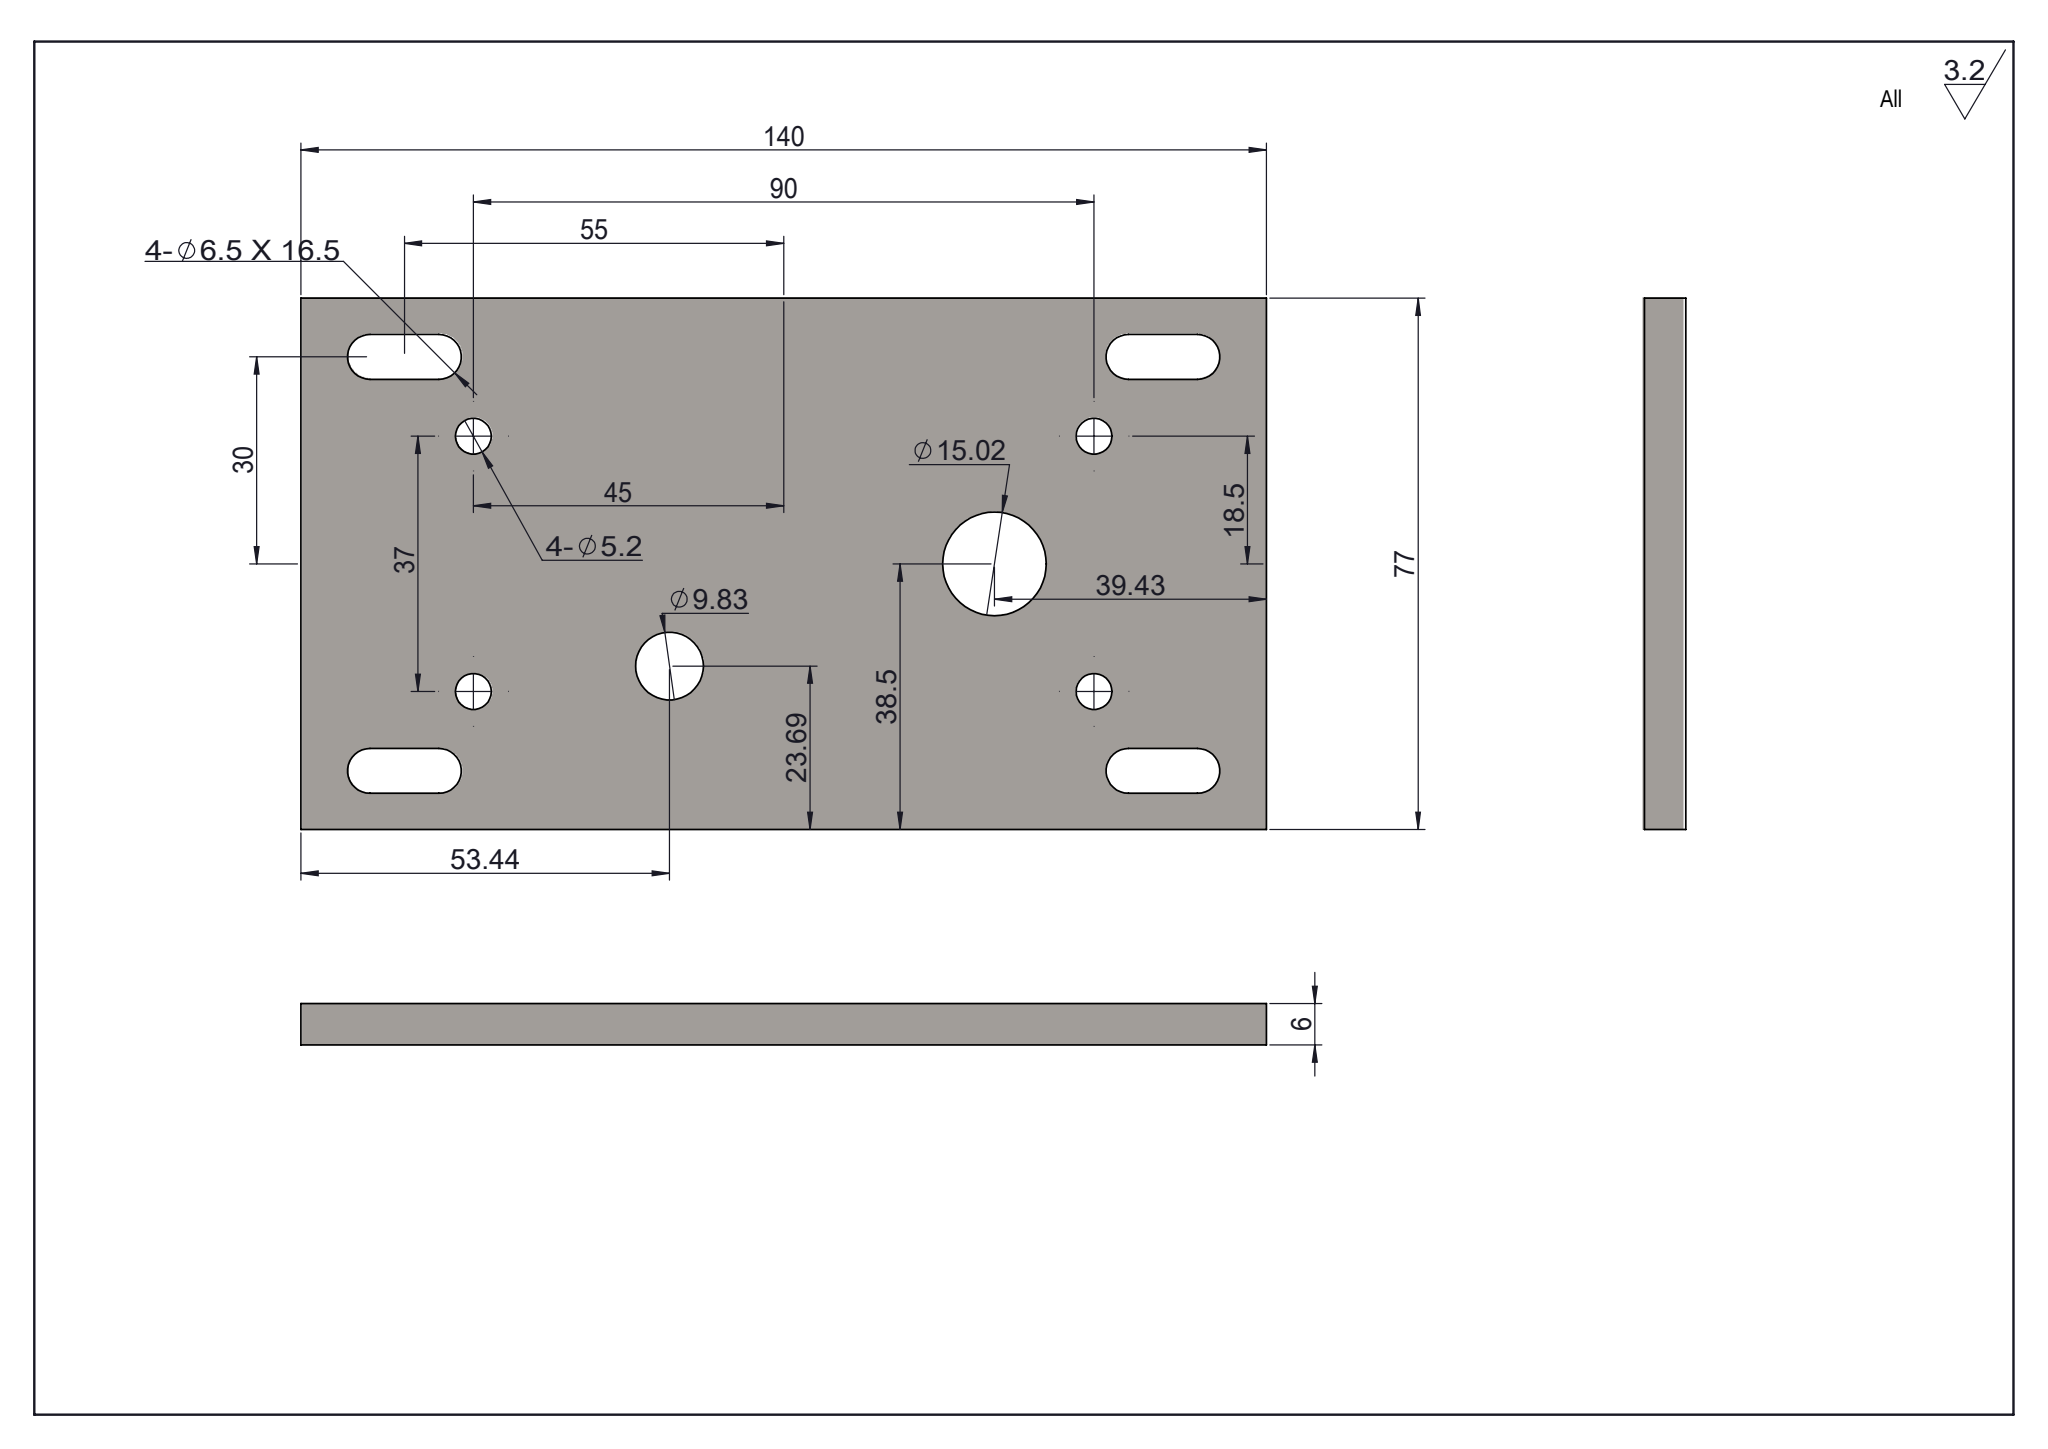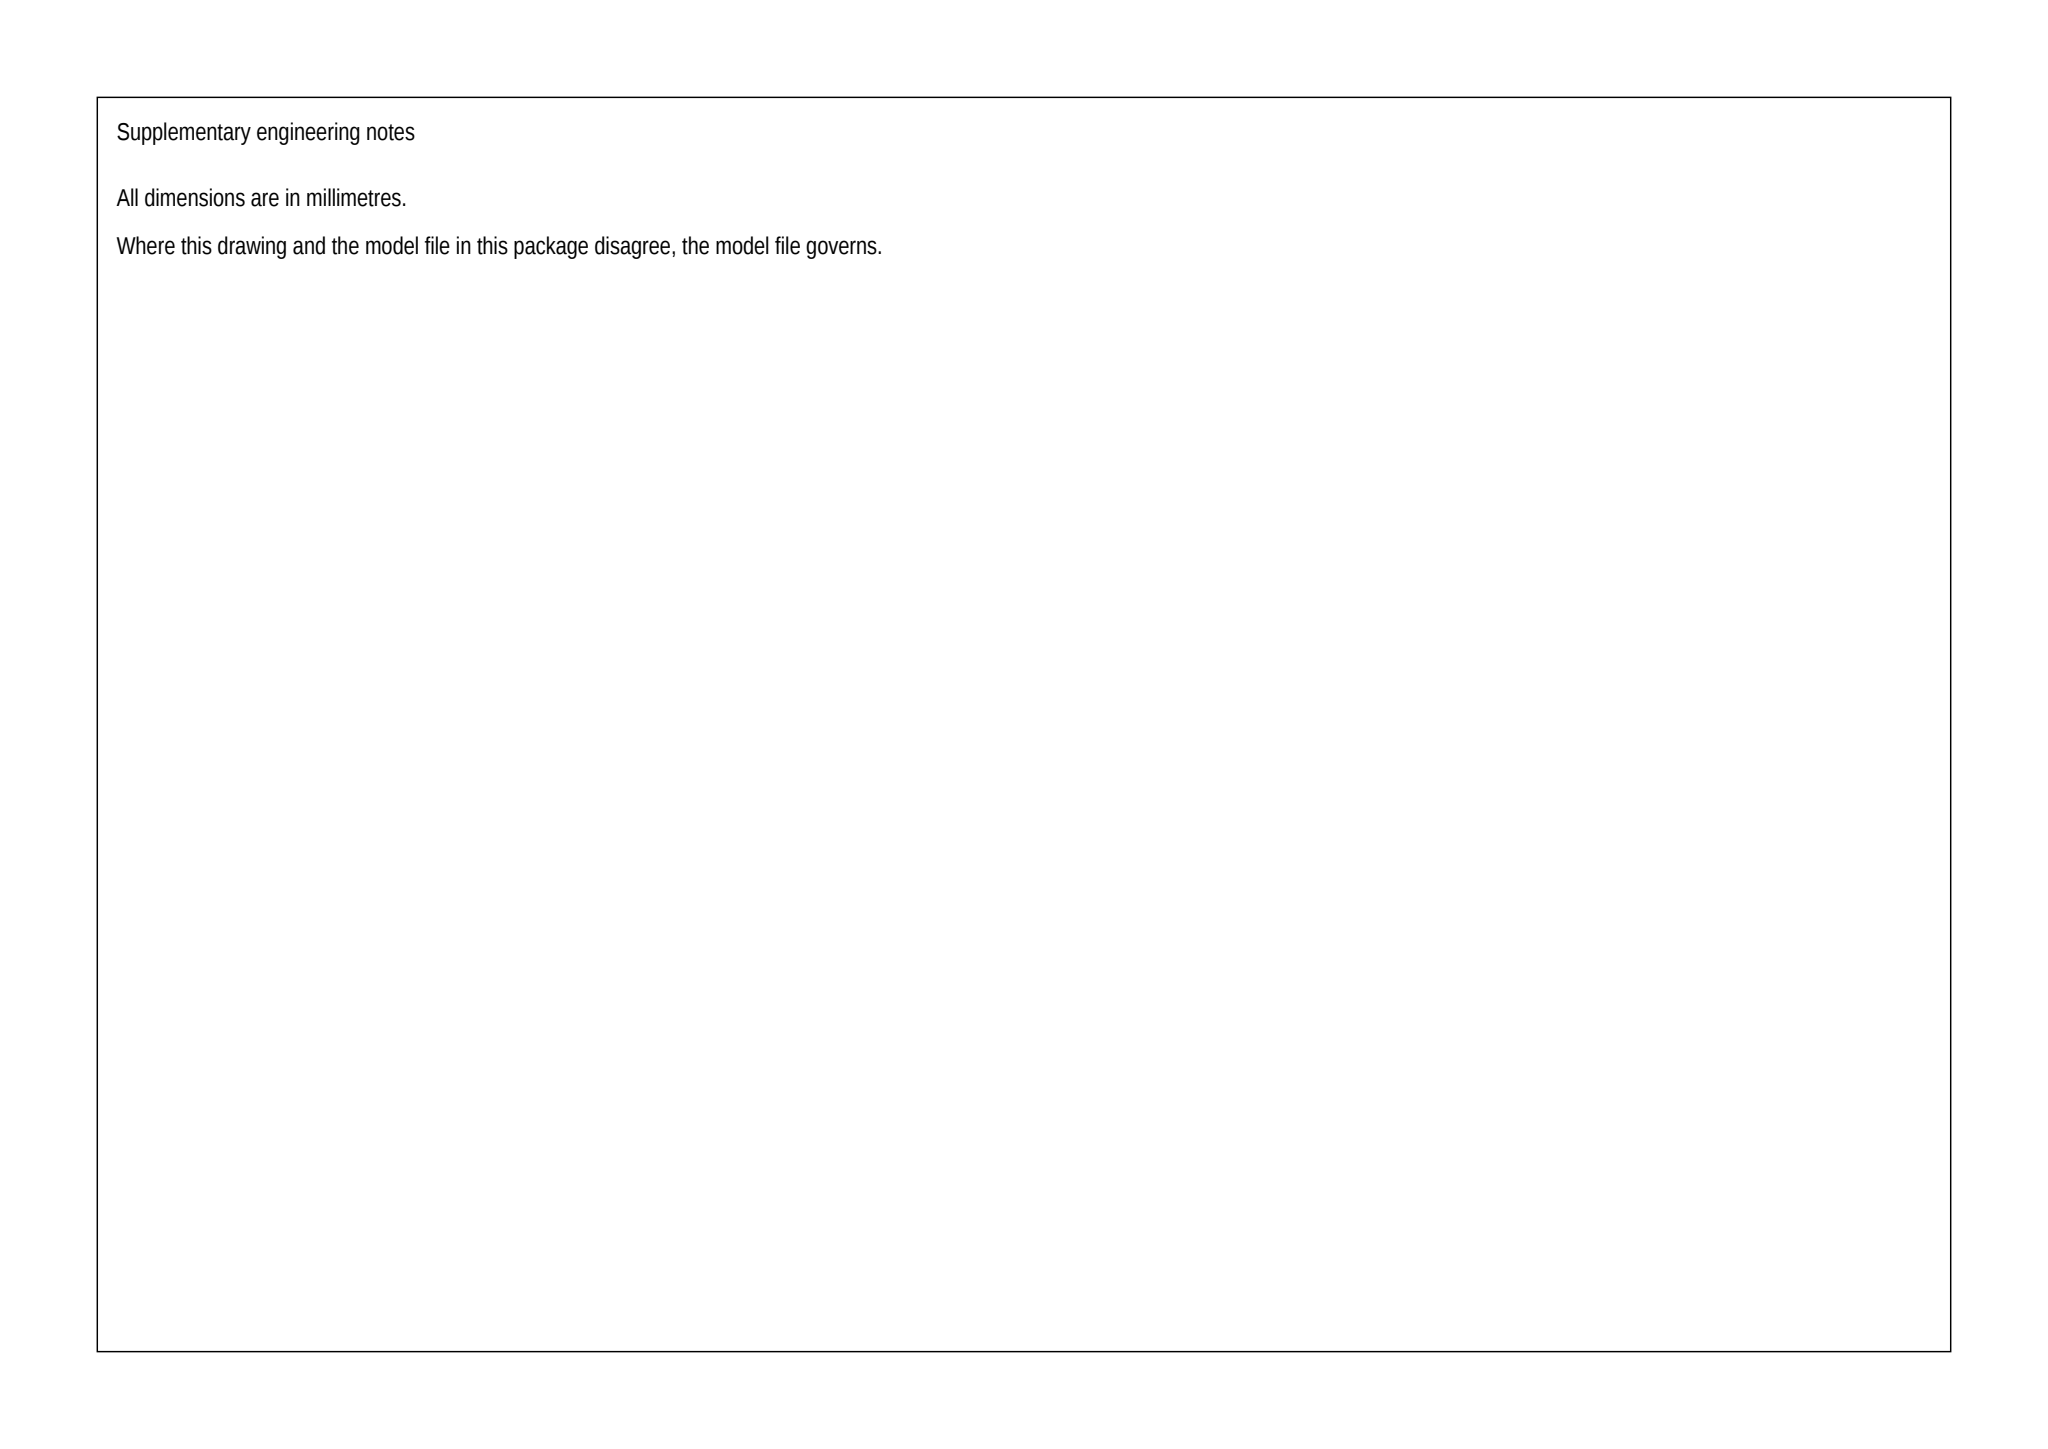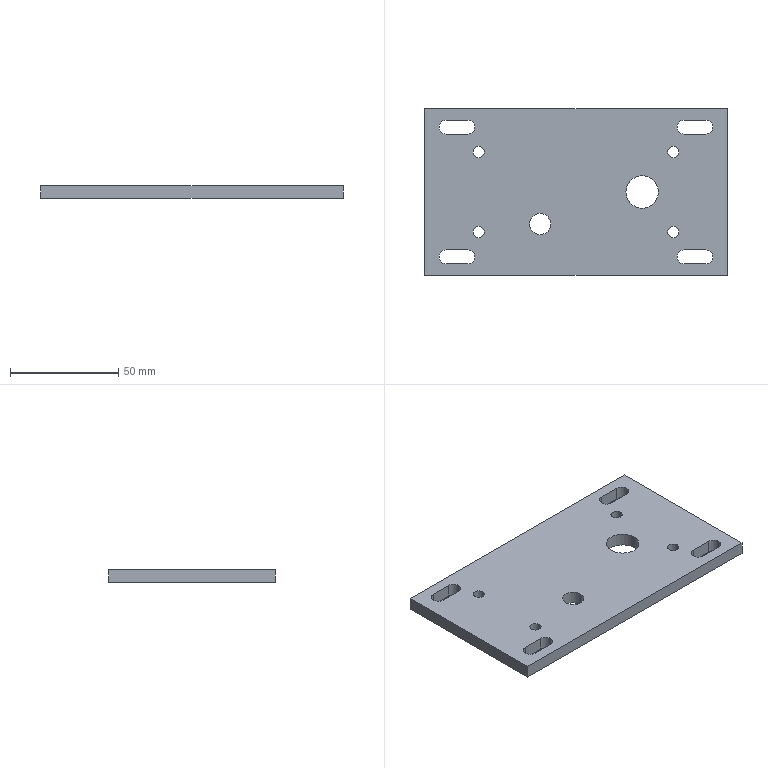Part | SolidWorks | mm | 1 solid | 38 faces | box 140 x 77 x 6 mm | volume 60295 mm3 | cylinder 24 | plane 14 | commonest cylinder face diameters 6.5 x12 5.2 x8 9.835 x2 15.02 x2
build123d program:
from build123d import *

# Parameters (mm, degrees)
SKETCH1_W           = 140
SKETCH1_H           = 77
BOSS_EXTRUDE1_DEPTH = 6
SKETCH3_R           = 2.6
CUT_EXTRUDE1_DEPTH  = 114.065
SKETCH4_R           = 4.917
SKETCH4_R_2         = 7.51
CUT_EXTRUDE2_DEPTH  = 80


with BuildPart() as part:
    # Sketch1 → Boss-Extrude1 (new body)
    with BuildSketch(Plane.XY):
        with Locations((-25.009, -22.5)):
            Rectangle(SKETCH1_W, SKETCH1_H)
    extrude(amount=BOSS_EXTRUDE1_DEPTH)

    # Sketch3 → Cut-Extrude1 (cut, through all)
    with BuildSketch(Plane.XY.offset(6)):
        with Locations((-70.009, -4)):
            Circle(SKETCH3_R)
        with Locations((19.991, -4)):
            Circle(SKETCH3_R)
        with Locations((-70.009, -41)):
            Circle(SKETCH3_R)
        with Locations((19.991, -41)):
            Circle(SKETCH3_R)
        with BuildLine():
            Line((-85.009, 10.75), (-75.009, 10.75))
            ThreePointArc((-75.009, 10.75), (-71.759, 7.5), (-75.009, 4.25))
            Line((-75.009, 4.25), (-85.009, 4.25))
            ThreePointArc((-85.009, 4.25), (-88.259, 7.5), (-85.009, 10.75))
        make_face()
        with BuildLine():
            Line((-85.009, -49.25), (-75.009, -49.25))
            ThreePointArc((-75.009, -49.25), (-71.759, -52.5), (-75.009, -55.75))
            Line((-75.009, -55.75), (-85.009, -55.75))
            ThreePointArc((-85.009, -55.75), (-88.259, -52.5), (-85.009, -49.25))
        make_face()
        with BuildLine():
            Line((24.991, 10.75), (34.991, 10.75))
            ThreePointArc((34.991, 10.75), (38.241, 7.5), (34.991, 4.25))
            Line((34.991, 4.25), (24.991, 4.25))
            ThreePointArc((24.991, 4.25), (21.741, 7.5), (24.991, 10.75))
        make_face()
        with BuildLine():
            Line((24.991, -49.25), (34.991, -49.25))
            ThreePointArc((34.991, -49.25), (38.241, -52.5), (34.991, -55.75))
            Line((34.991, -55.75), (24.991, -55.75))
            ThreePointArc((24.991, -55.75), (21.741, -52.5), (24.991, -49.25))
        make_face()
    extrude(amount=-CUT_EXTRUDE1_DEPTH, mode=Mode.SUBTRACT)

    # Sketch4 → Cut-Extrude2 (cut)
    with BuildSketch(Plane.XY.offset(6)):
        with Locations((-41.566, -37.306)):
            Circle(SKETCH4_R)
        with Locations((5.559, -22.5)):
            Circle(SKETCH4_R_2)
    extrude(amount=-CUT_EXTRUDE2_DEPTH, mode=Mode.SUBTRACT)


solid = part.part